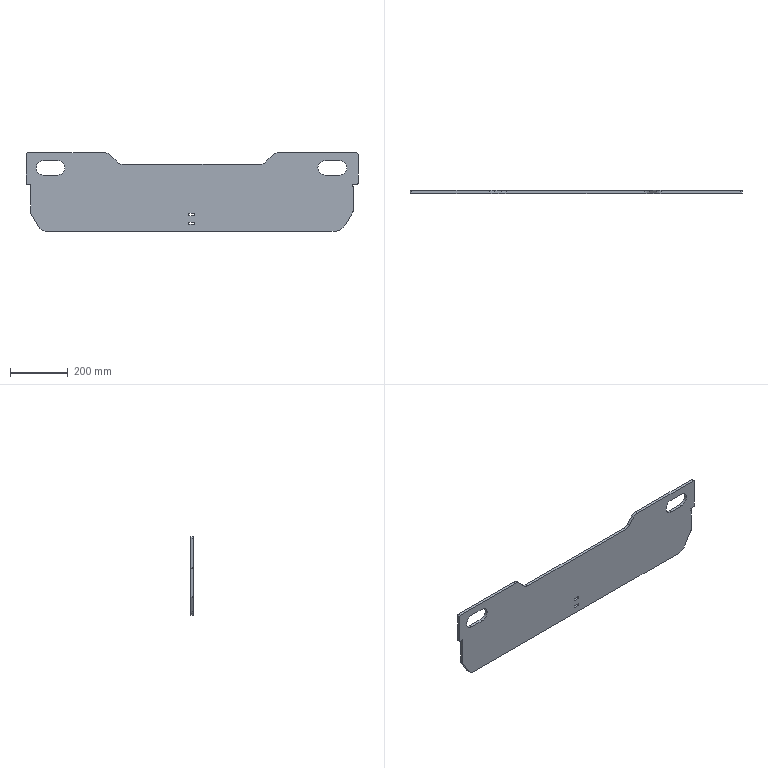Component | SolidWorks | FrontEndPlate-1 | 1 solid | 50 faces | volume 2741792 mm3 | plane 31 | cylinder 19 | commonest cylinder face diameters 50 x11 10 x6 80 x1 20 x1 | material Q235